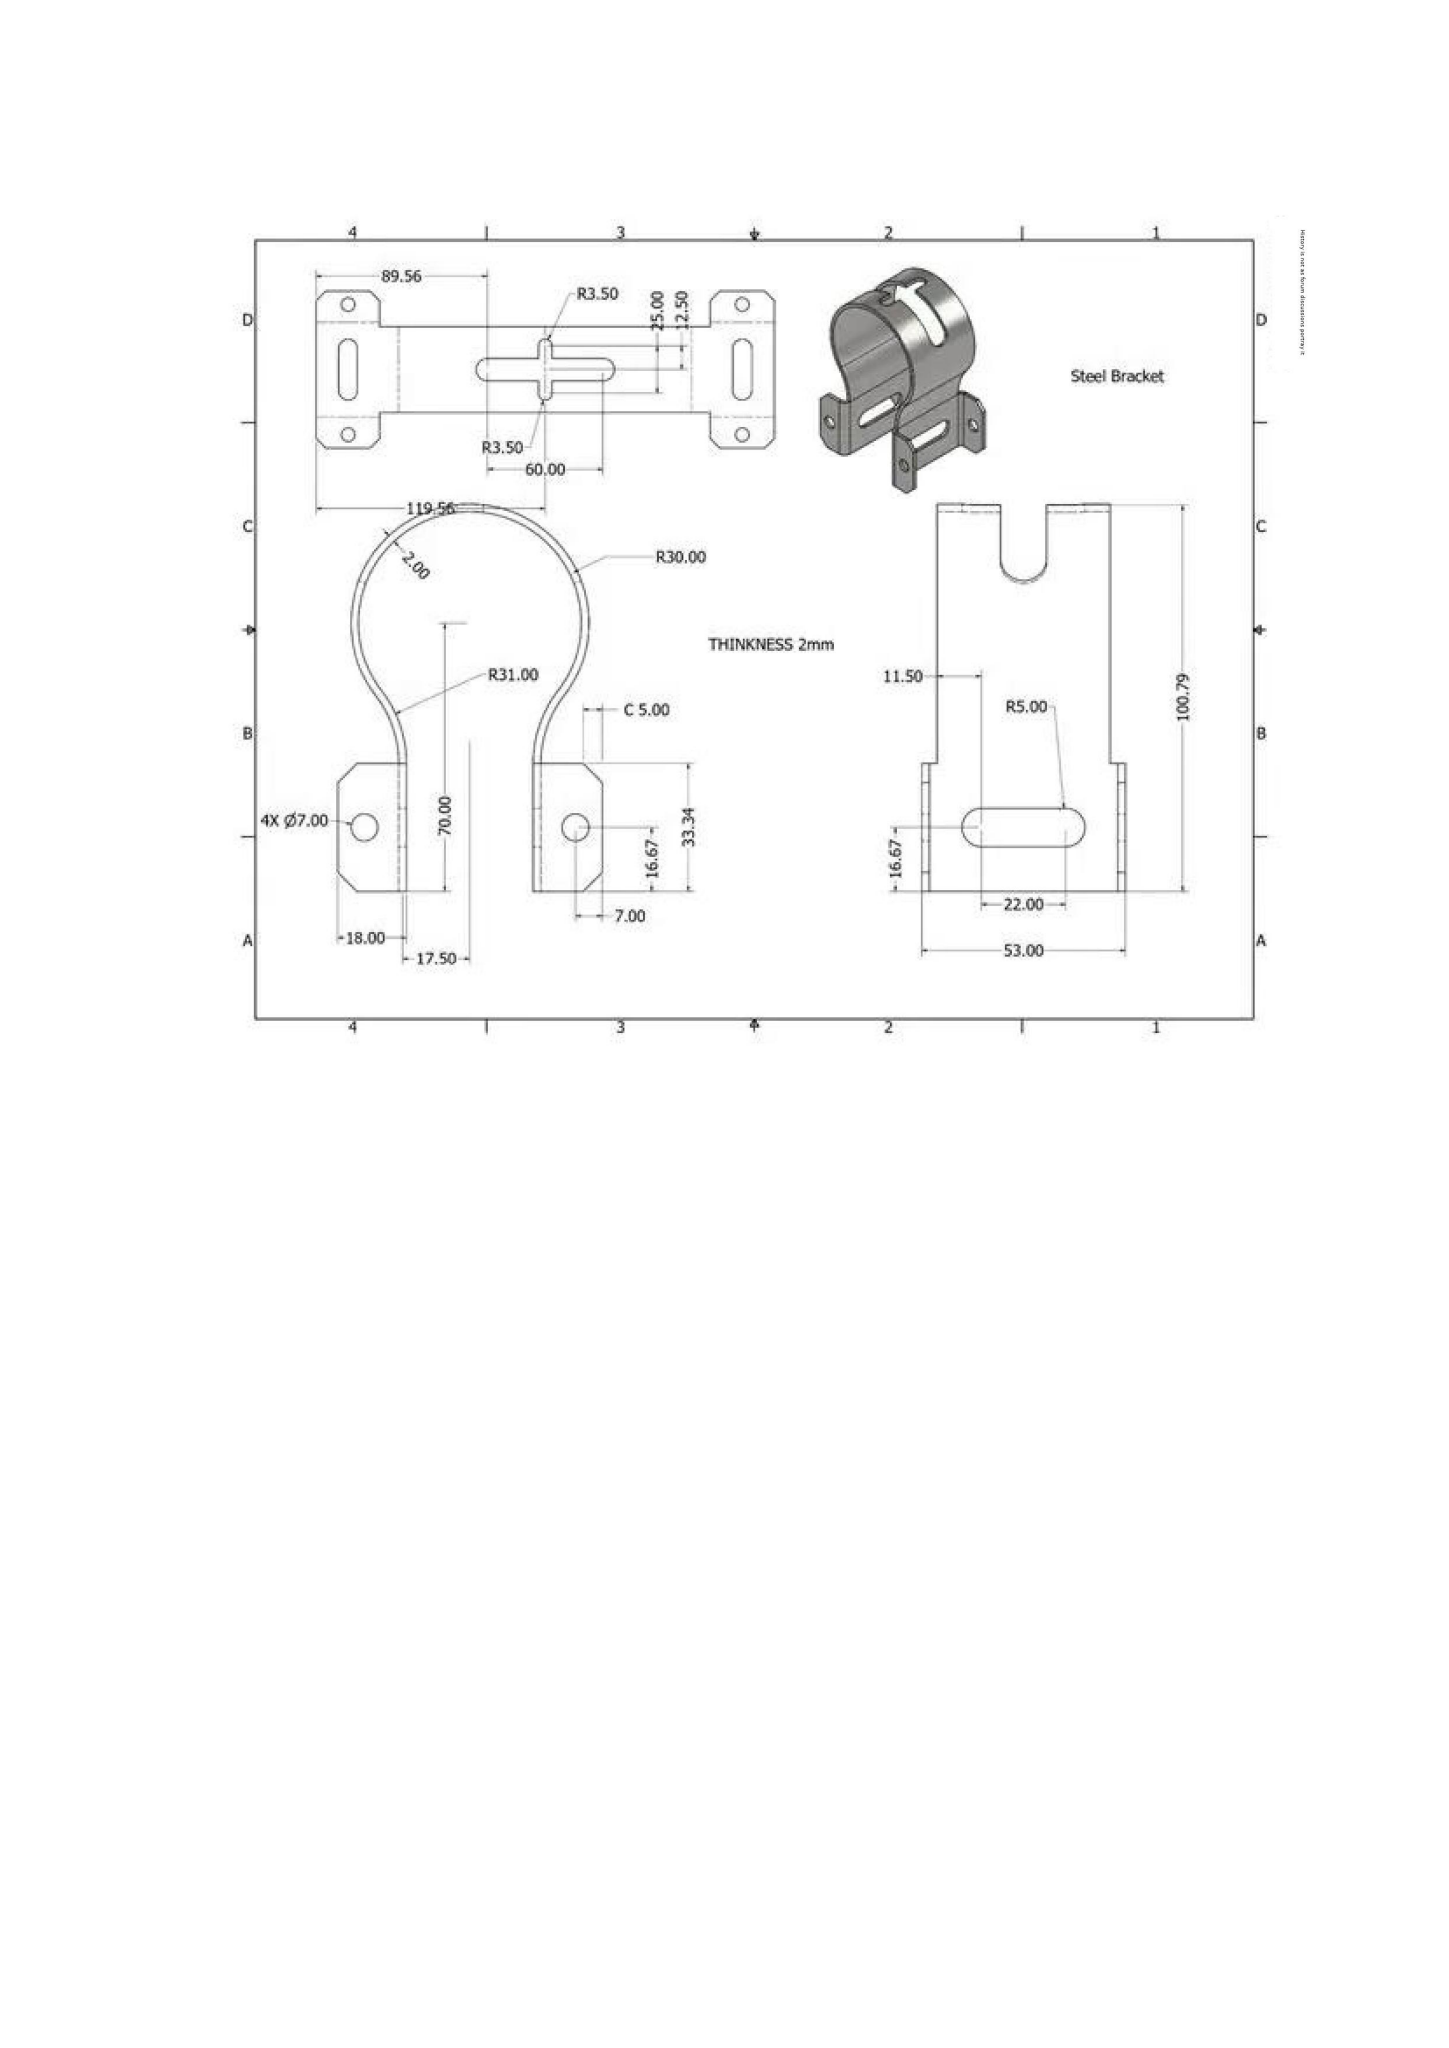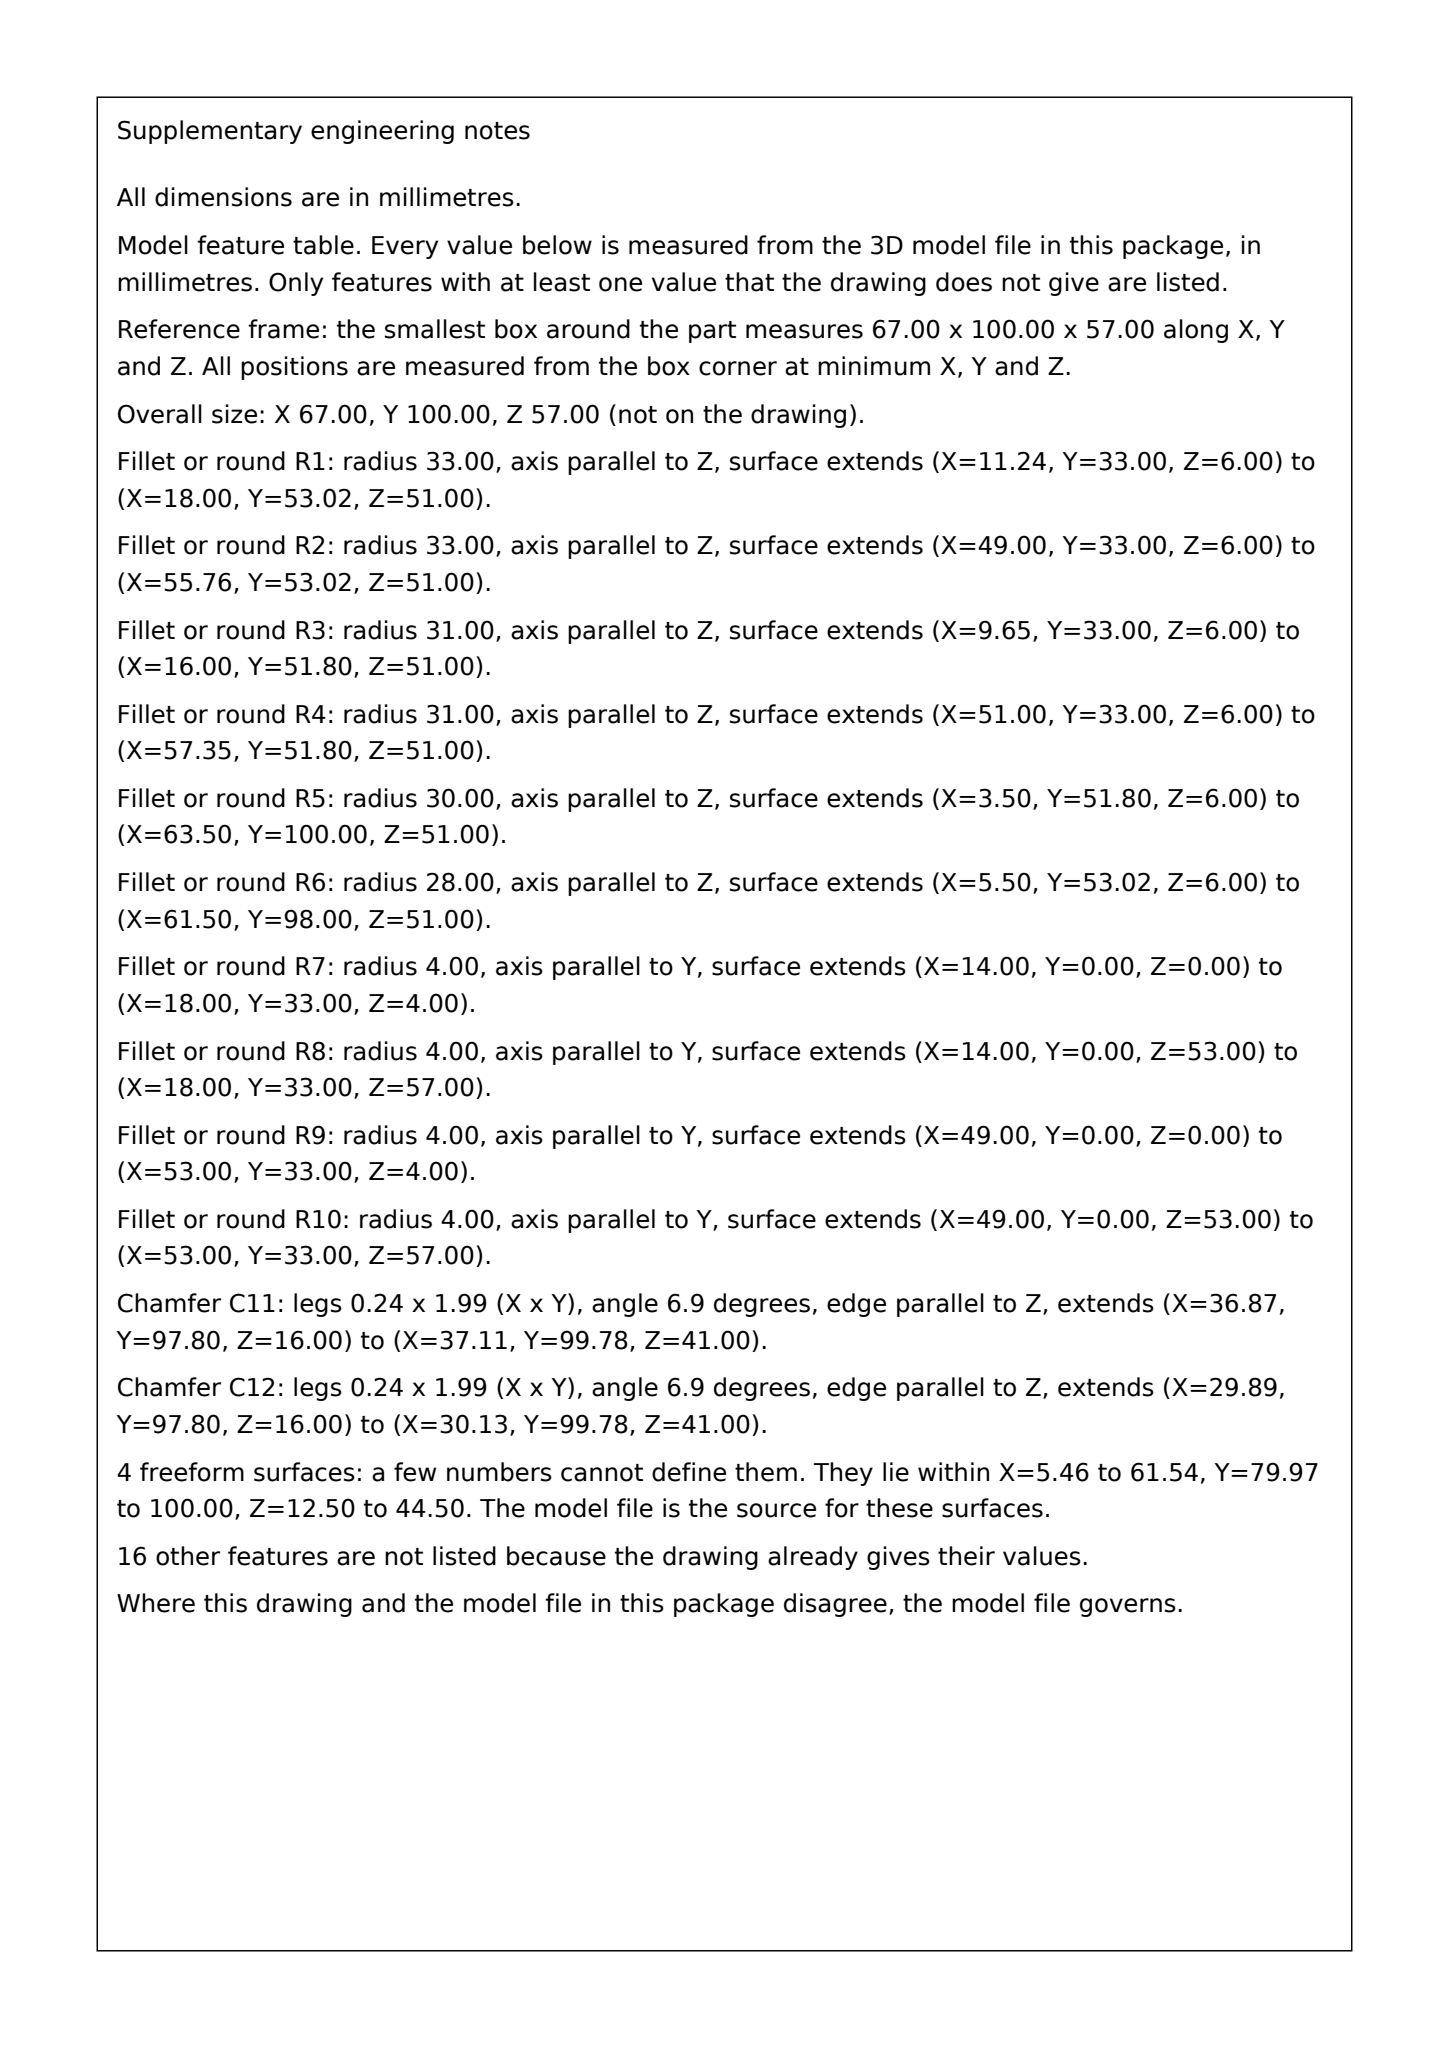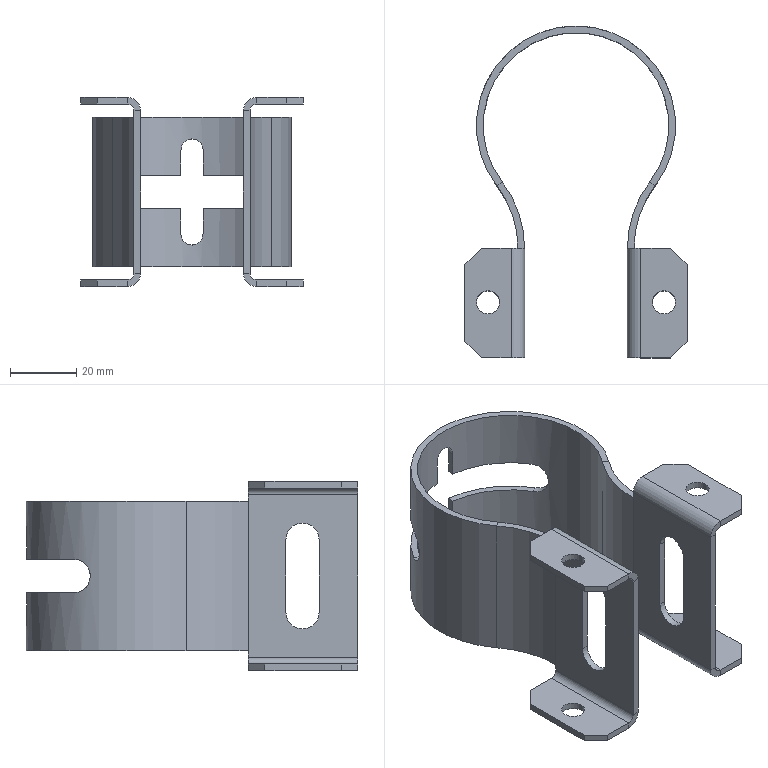Part | SolidWorks | mm | material Steel | 1 solid | 94 faces | box 67 x 100 x 57 mm | volume 23417 mm3 | plane 64 | cylinder 26 | spline 4 | commonest cylinder face diameters 7 x8 8 x4 4 x4 10 x4 62 x2 66 x2 60 x1 56 x1